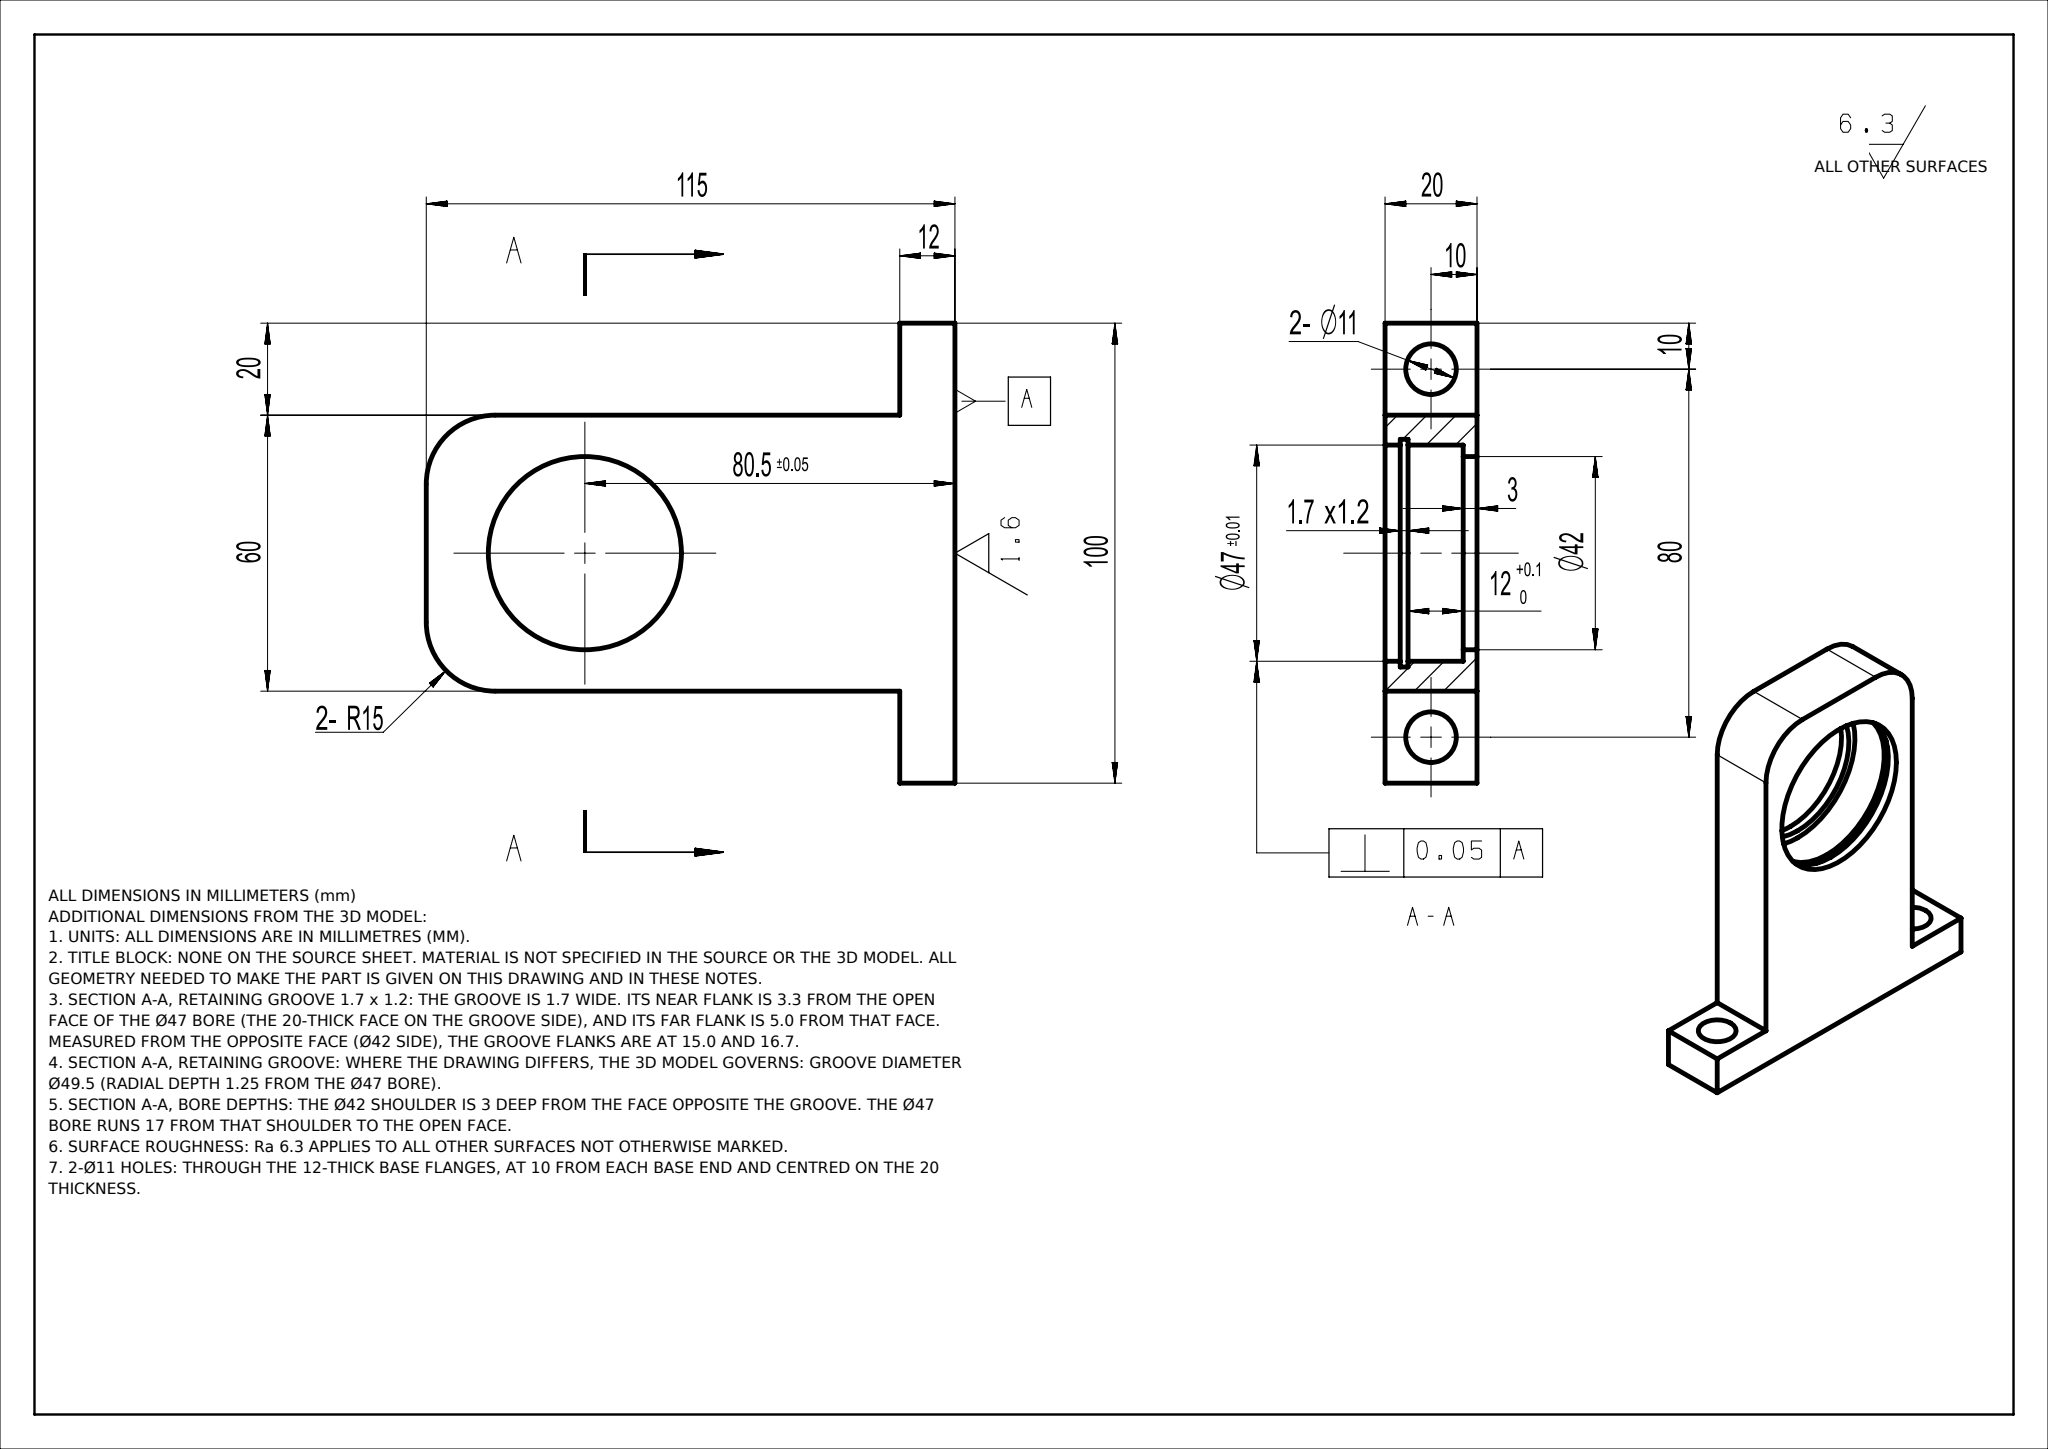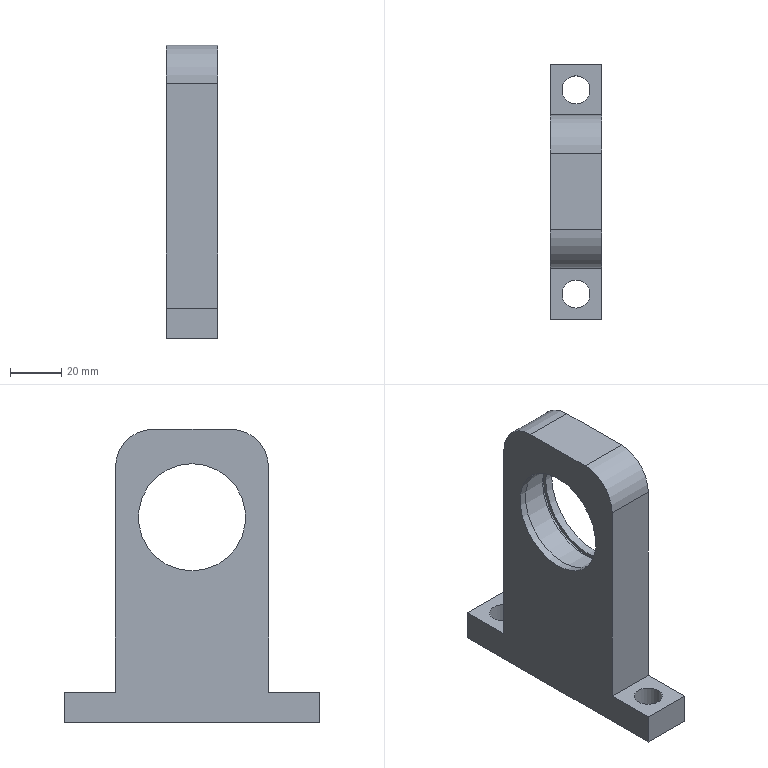Part | NX | mm | 1 solid | 21 faces | box 20 x 100 x 115 mm | volume 109415 mm3 | plane 13 | cylinder 8 | commonest cylinder face diameters 47 x2 11 x2 30 x2 42 x1 49.5 x1
STEP:
#1=CARTESIAN_POINT('',(0.,0.,0.));
#2=DIRECTION('',(0.,0.,1.));
#3=DIRECTION('',(1.,0.,0.));
#4=AXIS2_PLACEMENT_3D('',#1,#2,#3);
#5=(LENGTH_UNIT()NAMED_UNIT(*)SI_UNIT(.MILLI.,.METRE.));
#6=UNCERTAINTY_MEASURE_WITH_UNIT(LENGTH_MEASURE(0.00002),#5,'','');
#7=(NAMED_UNIT(*)PLANE_ANGLE_UNIT()SI_UNIT($,.RADIAN.));
#8=PLANE_ANGLE_MEASURE_WITH_UNIT(PLANE_ANGLE_MEASURE(0.01745),#7);
#9=DIMENSIONAL_EXPONENTS(0.,0.,0.,0.,0.,0.,0.);
#10=(CONVERSION_BASED_UNIT('',#8)NAMED_UNIT(#9)PLANE_ANGLE_UNIT());
#11=(NAMED_UNIT(*)SI_UNIT($,.STERADIAN.)SOLID_ANGLE_UNIT());
#12=(GEOMETRIC_REPRESENTATION_CONTEXT(3)GLOBAL_UNCERTAINTY_ASSIGNED_CONTEXT((#6))GLOBAL_UNIT_ASSIGNED_CONTEXT((#5,#10,#11))REPRESENTATION_CONTEXT('',''));
#13=SHAPE_REPRESENTATION('',(#4),#12);
#14=CARTESIAN_POINT('',(3.,50.,57.));
#15=VERTEX_POINT('',#14);
#16=CARTESIAN_POINT('',(3.,50.,80.5));
#17=DIRECTION('',(1.,0.,0.));
#18=DIRECTION('',(0.,0.,-1.));
#19=AXIS2_PLACEMENT_3D('',#16,#17,#18);
#20=CIRCLE('',#19,23.5);
#21=EDGE_CURVE('',#15,#15,#20,.T.);
#22=ORIENTED_EDGE('',*,*,#21,.F.);
#23=EDGE_LOOP('',(#22));
#24=FACE_BOUND('',#23,.T.);
#25=CARTESIAN_POINT('',(15.,50.,57.));
#26=VERTEX_POINT('',#25);
#27=CARTESIAN_POINT('',(15.,50.,80.5));
#28=DIRECTION('',(1.,0.,0.));
#29=DIRECTION('',(0.,0.,-1.));
#30=AXIS2_PLACEMENT_3D('',#27,#28,#29);
#31=CIRCLE('',#30,23.5);
#32=EDGE_CURVE('',#26,#26,#31,.T.);
#33=ORIENTED_EDGE('',*,*,#32,.T.);
#34=EDGE_LOOP('',(#33));
#35=FACE_BOUND('',#34,.T.);
#36=CARTESIAN_POINT('',(20.,50.,80.5));
#37=DIRECTION('',(-1.,0.,0.));
#38=DIRECTION('',(0.,0.,1.));
#39=AXIS2_PLACEMENT_3D('',#36,#37,#38);
#40=CYLINDRICAL_SURFACE('',#39,23.5);
#41=ADVANCED_FACE('',(#24,#35),#40,.F.);
#42=CARTESIAN_POINT('',(0.,-0.,0.));
#43=VERTEX_POINT('',#42);
#44=CARTESIAN_POINT('',(0.,100.,0.));
#45=VERTEX_POINT('',#44);
#46=CARTESIAN_POINT('',(0.,0.,0.));
#47=DIRECTION('',(0.,1.,0.));
#48=VECTOR('',#47,1.);
#49=LINE('',#46,#48);
#50=EDGE_CURVE('',#43,#45,#49,.T.);
#51=ORIENTED_EDGE('',*,*,#50,.T.);
#52=CARTESIAN_POINT('',(20.,100.,0.));
#53=VERTEX_POINT('',#52);
#54=CARTESIAN_POINT('',(20.,100.,0.));
#55=DIRECTION('',(-1.,0.,0.));
#56=VECTOR('',#55,1.);
#57=LINE('',#54,#56);
#58=EDGE_CURVE('',#53,#45,#57,.T.);
#59=ORIENTED_EDGE('',*,*,#58,.F.);
#60=CARTESIAN_POINT('',(20.,-0.,0.));
#61=VERTEX_POINT('',#60);
#62=CARTESIAN_POINT('',(20.,0.,0.));
#63=DIRECTION('',(0.,1.,0.));
#64=VECTOR('',#63,1.);
#65=LINE('',#62,#64);
#66=EDGE_CURVE('',#61,#53,#65,.T.);
#67=ORIENTED_EDGE('',*,*,#66,.F.);
#68=CARTESIAN_POINT('',(20.,-0.,0.));
#69=DIRECTION('',(-1.,0.,0.));
#70=VECTOR('',#69,1.);
#71=LINE('',#68,#70);
#72=EDGE_CURVE('',#61,#43,#71,.T.);
#73=ORIENTED_EDGE('',*,*,#72,.T.);
#74=EDGE_LOOP('',(#51,#59,#67,#73));
#75=FACE_BOUND('',#74,.T.);
#76=CARTESIAN_POINT('',(10.,15.5,0.));
#77=VERTEX_POINT('',#76);
#78=CARTESIAN_POINT('',(10.,10.,0.));
#79=DIRECTION('',(0.,0.,-1.));
#80=DIRECTION('',(0.,1.,0.));
#81=AXIS2_PLACEMENT_3D('',#78,#79,#80);
#82=CIRCLE('',#81,5.5);
#83=EDGE_CURVE('',#77,#77,#82,.T.);
#84=ORIENTED_EDGE('',*,*,#83,.F.);
#85=EDGE_LOOP('',(#84));
#86=FACE_BOUND('',#85,.T.);
#87=CARTESIAN_POINT('',(10.,84.5,0.));
#88=VERTEX_POINT('',#87);
#89=CARTESIAN_POINT('',(10.,90.,0.));
#90=DIRECTION('',(0.,0.,1.));
#91=DIRECTION('',(-0.,-1.,0.));
#92=AXIS2_PLACEMENT_3D('',#89,#90,#91);
#93=CIRCLE('',#92,5.5);
#94=EDGE_CURVE('',#88,#88,#93,.T.);
#95=ORIENTED_EDGE('',*,*,#94,.T.);
#96=EDGE_LOOP('',(#95));
#97=FACE_BOUND('',#96,.T.);
#98=CARTESIAN_POINT('',(20.,0.,0.));
#99=DIRECTION('',(0.,0.,1.));
#100=DIRECTION('',(1.,0.,0.));
#101=AXIS2_PLACEMENT_3D('',#98,#99,#100);
#102=PLANE('',#101);
#103=ADVANCED_FACE('',(#75,#86,#97),#102,.F.);
#104=CARTESIAN_POINT('',(0.,0.,12.));
#105=VERTEX_POINT('',#104);
#106=CARTESIAN_POINT('',(0.,0.,12.));
#107=DIRECTION('',(0.,-0.,-1.));
#108=VECTOR('',#107,1.);
#109=LINE('',#106,#108);
#110=EDGE_CURVE('',#105,#43,#109,.T.);
#111=ORIENTED_EDGE('',*,*,#110,.T.);
#112=ORIENTED_EDGE('',*,*,#72,.F.);
#113=CARTESIAN_POINT('',(20.,0.,12.));
#114=VERTEX_POINT('',#113);
#115=CARTESIAN_POINT('',(20.,0.,12.));
#116=DIRECTION('',(0.,-0.,-1.));
#117=VECTOR('',#116,1.);
#118=LINE('',#115,#117);
#119=EDGE_CURVE('',#114,#61,#118,.T.);
#120=ORIENTED_EDGE('',*,*,#119,.F.);
#121=CARTESIAN_POINT('',(20.,0.,12.));
#122=DIRECTION('',(-1.,0.,0.));
#123=VECTOR('',#122,1.);
#124=LINE('',#121,#123);
#125=EDGE_CURVE('',#114,#105,#124,.T.);
#126=ORIENTED_EDGE('',*,*,#125,.T.);
#127=EDGE_LOOP('',(#111,#112,#120,#126));
#128=FACE_OUTER_BOUND('',#127,.T.);
#129=CARTESIAN_POINT('',(20.,0.,12.));
#130=DIRECTION('',(0.,1.,-0.));
#131=DIRECTION('',(0.,0.,1.));
#132=AXIS2_PLACEMENT_3D('',#129,#130,#131);
#133=PLANE('',#132);
#134=ADVANCED_FACE('',(#128),#133,.F.);
#135=CARTESIAN_POINT('',(0.,100.,12.));
#136=VERTEX_POINT('',#135);
#137=CARTESIAN_POINT('',(0.,100.,0.));
#138=DIRECTION('',(0.,0.,1.));
#139=VECTOR('',#138,1.);
#140=LINE('',#137,#139);
#141=EDGE_CURVE('',#45,#136,#140,.T.);
#142=ORIENTED_EDGE('',*,*,#141,.T.);
#143=CARTESIAN_POINT('',(20.,100.,12.));
#144=VERTEX_POINT('',#143);
#145=CARTESIAN_POINT('',(20.,100.,12.));
#146=DIRECTION('',(-1.,0.,0.));
#147=VECTOR('',#146,1.);
#148=LINE('',#145,#147);
#149=EDGE_CURVE('',#144,#136,#148,.T.);
#150=ORIENTED_EDGE('',*,*,#149,.F.);
#151=CARTESIAN_POINT('',(20.,100.,0.));
#152=DIRECTION('',(0.,0.,1.));
#153=VECTOR('',#152,1.);
#154=LINE('',#151,#153);
#155=EDGE_CURVE('',#53,#144,#154,.T.);
#156=ORIENTED_EDGE('',*,*,#155,.F.);
#157=ORIENTED_EDGE('',*,*,#58,.T.);
#158=EDGE_LOOP('',(#142,#150,#156,#157));
#159=FACE_OUTER_BOUND('',#158,.T.);
#160=CARTESIAN_POINT('',(20.,100.,0.));
#161=DIRECTION('',(0.,-1.,0.));
#162=DIRECTION('',(0.,0.,-1.));
#163=AXIS2_PLACEMENT_3D('',#160,#161,#162);
#164=PLANE('',#163);
#165=ADVANCED_FACE('',(#159),#164,.F.);
#166=CARTESIAN_POINT('',(10.,95.5,12.));
#167=VERTEX_POINT('',#166);
#168=CARTESIAN_POINT('',(10.,90.,12.));
#169=DIRECTION('',(0.,-0.,1.));
#170=DIRECTION('',(0.,1.,0.));
#171=AXIS2_PLACEMENT_3D('',#168,#169,#170);
#172=CIRCLE('',#171,5.5);
#173=EDGE_CURVE('',#167,#167,#172,.T.);
#174=ORIENTED_EDGE('',*,*,#173,.F.);
#175=EDGE_LOOP('',(#174));
#176=FACE_BOUND('',#175,.T.);
#177=CARTESIAN_POINT('',(0.,80.,12.));
#178=VERTEX_POINT('',#177);
#179=CARTESIAN_POINT('',(0.,100.,12.));
#180=DIRECTION('',(0.,-1.,-0.));
#181=VECTOR('',#180,1.);
#182=LINE('',#179,#181);
#183=EDGE_CURVE('',#136,#178,#182,.T.);
#184=ORIENTED_EDGE('',*,*,#183,.T.);
#185=CARTESIAN_POINT('',(20.,80.,12.));
#186=VERTEX_POINT('',#185);
#187=CARTESIAN_POINT('',(20.,80.,12.));
#188=DIRECTION('',(-1.,0.,0.));
#189=VECTOR('',#188,1.);
#190=LINE('',#187,#189);
#191=EDGE_CURVE('',#186,#178,#190,.T.);
#192=ORIENTED_EDGE('',*,*,#191,.F.);
#193=CARTESIAN_POINT('',(20.,100.,12.));
#194=DIRECTION('',(0.,-1.,-0.));
#195=VECTOR('',#194,1.);
#196=LINE('',#193,#195);
#197=EDGE_CURVE('',#144,#186,#196,.T.);
#198=ORIENTED_EDGE('',*,*,#197,.F.);
#199=ORIENTED_EDGE('',*,*,#149,.T.);
#200=EDGE_LOOP('',(#184,#192,#198,#199));
#201=FACE_BOUND('',#200,.T.);
#202=CARTESIAN_POINT('',(20.,100.,12.));
#203=DIRECTION('',(0.,0.,-1.));
#204=DIRECTION('',(0.,1.,0.));
#205=AXIS2_PLACEMENT_3D('',#202,#203,#204);
#206=PLANE('',#205);
#207=ADVANCED_FACE('',(#176,#201),#206,.F.);
#208=CARTESIAN_POINT('',(0.,80.,100.));
#209=VERTEX_POINT('',#208);
#210=CARTESIAN_POINT('',(0.,80.,12.));
#211=DIRECTION('',(0.,-0.,1.));
#212=VECTOR('',#211,1.);
#213=LINE('',#210,#212);
#214=EDGE_CURVE('',#178,#209,#213,.T.);
#215=ORIENTED_EDGE('',*,*,#214,.T.);
#216=CARTESIAN_POINT('',(20.,80.,100.));
#217=VERTEX_POINT('',#216);
#218=CARTESIAN_POINT('',(20.,80.,100.));
#219=DIRECTION('',(1.,0.,0.));
#220=VECTOR('',#219,1.);
#221=LINE('',#218,#220);
#222=EDGE_CURVE('',#209,#217,#221,.T.);
#223=ORIENTED_EDGE('',*,*,#222,.T.);
#224=CARTESIAN_POINT('',(20.,80.,12.));
#225=DIRECTION('',(0.,-0.,1.));
#226=VECTOR('',#225,1.);
#227=LINE('',#224,#226);
#228=EDGE_CURVE('',#186,#217,#227,.T.);
#229=ORIENTED_EDGE('',*,*,#228,.F.);
#230=ORIENTED_EDGE('',*,*,#191,.T.);
#231=EDGE_LOOP('',(#215,#223,#229,#230));
#232=FACE_OUTER_BOUND('',#231,.T.);
#233=CARTESIAN_POINT('',(20.,80.,12.));
#234=DIRECTION('',(0.,-1.,-0.));
#235=DIRECTION('',(0.,0.,-1.));
#236=AXIS2_PLACEMENT_3D('',#233,#234,#235);
#237=PLANE('',#236);
#238=ADVANCED_FACE('',(#232),#237,.F.);
#239=CARTESIAN_POINT('',(20.,65.,115.));
#240=VERTEX_POINT('',#239);
#241=CARTESIAN_POINT('',(20.,35.,115.));
#242=VERTEX_POINT('',#241);
#243=CARTESIAN_POINT('',(20.,80.,115.));
#244=DIRECTION('',(0.,-1.,-0.));
#245=VECTOR('',#244,1.);
#246=LINE('',#243,#245);
#247=EDGE_CURVE('',#240,#242,#246,.T.);
#248=ORIENTED_EDGE('',*,*,#247,.F.);
#249=CARTESIAN_POINT('',(0.,65.,115.));
#250=VERTEX_POINT('',#249);
#251=CARTESIAN_POINT('',(20.,65.,115.));
#252=DIRECTION('',(-1.,0.,0.));
#253=VECTOR('',#252,1.);
#254=LINE('',#251,#253);
#255=EDGE_CURVE('',#240,#250,#254,.T.);
#256=ORIENTED_EDGE('',*,*,#255,.T.);
#257=CARTESIAN_POINT('',(0.,35.,115.));
#258=VERTEX_POINT('',#257);
#259=CARTESIAN_POINT('',(0.,80.,115.));
#260=DIRECTION('',(0.,-1.,-0.));
#261=VECTOR('',#260,1.);
#262=LINE('',#259,#261);
#263=EDGE_CURVE('',#250,#258,#262,.T.);
#264=ORIENTED_EDGE('',*,*,#263,.T.);
#265=CARTESIAN_POINT('',(20.,35.,115.));
#266=DIRECTION('',(1.,0.,0.));
#267=VECTOR('',#266,1.);
#268=LINE('',#265,#267);
#269=EDGE_CURVE('',#258,#242,#268,.T.);
#270=ORIENTED_EDGE('',*,*,#269,.T.);
#271=EDGE_LOOP('',(#248,#256,#264,#270));
#272=FACE_OUTER_BOUND('',#271,.T.);
#273=CARTESIAN_POINT('',(20.,80.,115.));
#274=DIRECTION('',(0.,0.,-1.));
#275=DIRECTION('',(0.,1.,0.));
#276=AXIS2_PLACEMENT_3D('',#273,#274,#275);
#277=PLANE('',#276);
#278=ADVANCED_FACE('',(#272),#277,.F.);
#279=CARTESIAN_POINT('',(20.,20.,100.));
#280=VERTEX_POINT('',#279);
#281=CARTESIAN_POINT('',(20.,20.,12.));
#282=VERTEX_POINT('',#281);
#283=CARTESIAN_POINT('',(20.,20.,115.));
#284=DIRECTION('',(0.,0.,-1.));
#285=VECTOR('',#284,1.);
#286=LINE('',#283,#285);
#287=EDGE_CURVE('',#280,#282,#286,.T.);
#288=ORIENTED_EDGE('',*,*,#287,.F.);
#289=CARTESIAN_POINT('',(0.,20.,100.));
#290=VERTEX_POINT('',#289);
#291=CARTESIAN_POINT('',(20.,20.,100.));
#292=DIRECTION('',(-1.,0.,0.));
#293=VECTOR('',#292,1.);
#294=LINE('',#291,#293);
#295=EDGE_CURVE('',#280,#290,#294,.T.);
#296=ORIENTED_EDGE('',*,*,#295,.T.);
#297=CARTESIAN_POINT('',(0.,20.,12.));
#298=VERTEX_POINT('',#297);
#299=CARTESIAN_POINT('',(0.,20.,115.));
#300=DIRECTION('',(0.,0.,-1.));
#301=VECTOR('',#300,1.);
#302=LINE('',#299,#301);
#303=EDGE_CURVE('',#290,#298,#302,.T.);
#304=ORIENTED_EDGE('',*,*,#303,.T.);
#305=CARTESIAN_POINT('',(20.,20.,12.));
#306=DIRECTION('',(-1.,0.,0.));
#307=VECTOR('',#306,1.);
#308=LINE('',#305,#307);
#309=EDGE_CURVE('',#282,#298,#308,.T.);
#310=ORIENTED_EDGE('',*,*,#309,.F.);
#311=EDGE_LOOP('',(#288,#296,#304,#310));
#312=FACE_OUTER_BOUND('',#311,.T.);
#313=CARTESIAN_POINT('',(20.,20.,115.));
#314=DIRECTION('',(0.,1.,0.));
#315=DIRECTION('',(0.,-0.,1.));
#316=AXIS2_PLACEMENT_3D('',#313,#314,#315);
#317=PLANE('',#316);
#318=ADVANCED_FACE('',(#312),#317,.F.);
#319=CARTESIAN_POINT('',(10.,15.5,12.));
#320=VERTEX_POINT('',#319);
#321=CARTESIAN_POINT('',(10.,10.,12.));
#322=DIRECTION('',(0.,0.,-1.));
#323=DIRECTION('',(0.,1.,0.));
#324=AXIS2_PLACEMENT_3D('',#321,#322,#323);
#325=CIRCLE('',#324,5.5);
#326=EDGE_CURVE('',#320,#320,#325,.T.);
#327=ORIENTED_EDGE('',*,*,#326,.T.);
#328=EDGE_LOOP('',(#327));
#329=FACE_BOUND('',#328,.T.);
#330=CARTESIAN_POINT('',(0.,20.,12.));
#331=DIRECTION('',(0.,-1.,-0.));
#332=VECTOR('',#331,1.);
#333=LINE('',#330,#332);
#334=EDGE_CURVE('',#298,#105,#333,.T.);
#335=ORIENTED_EDGE('',*,*,#334,.T.);
#336=ORIENTED_EDGE('',*,*,#125,.F.);
#337=CARTESIAN_POINT('',(20.,20.,12.));
#338=DIRECTION('',(0.,-1.,-0.));
#339=VECTOR('',#338,1.);
#340=LINE('',#337,#339);
#341=EDGE_CURVE('',#282,#114,#340,.T.);
#342=ORIENTED_EDGE('',*,*,#341,.F.);
#343=ORIENTED_EDGE('',*,*,#309,.T.);
#344=EDGE_LOOP('',(#335,#336,#342,#343));
#345=FACE_BOUND('',#344,.T.);
#346=CARTESIAN_POINT('',(20.,20.,12.));
#347=DIRECTION('',(0.,0.,-1.));
#348=DIRECTION('',(0.,1.,0.));
#349=AXIS2_PLACEMENT_3D('',#346,#347,#348);
#350=PLANE('',#349);
#351=ADVANCED_FACE('',(#329,#345),#350,.F.);
#352=CARTESIAN_POINT('',(16.7,50.,57.));
#353=VERTEX_POINT('',#352);
#354=CARTESIAN_POINT('',(16.7,50.,80.5));
#355=DIRECTION('',(1.,0.,0.));
#356=DIRECTION('',(0.,0.,-1.));
#357=AXIS2_PLACEMENT_3D('',#354,#355,#356);
#358=CIRCLE('',#357,23.5);
#359=EDGE_CURVE('',#353,#353,#358,.T.);
#360=ORIENTED_EDGE('',*,*,#359,.F.);
#361=EDGE_LOOP('',(#360));
#362=FACE_BOUND('',#361,.T.);
#363=CARTESIAN_POINT('',(20.,73.5,80.5));
#364=VERTEX_POINT('',#363);
#365=CARTESIAN_POINT('',(20.,50.,80.5));
#366=DIRECTION('',(1.,0.,0.));
#367=DIRECTION('',(0.,1.,0.));
#368=AXIS2_PLACEMENT_3D('',#365,#366,#367);
#369=CIRCLE('',#368,23.5);
#370=EDGE_CURVE('',#364,#364,#369,.T.);
#371=ORIENTED_EDGE('',*,*,#370,.T.);
#372=EDGE_LOOP('',(#371));
#373=FACE_BOUND('',#372,.T.);
#374=CARTESIAN_POINT('',(20.,50.,80.5));
#375=DIRECTION('',(-1.,0.,0.));
#376=DIRECTION('',(0.,0.,1.));
#377=AXIS2_PLACEMENT_3D('',#374,#375,#376);
#378=CYLINDRICAL_SURFACE('',#377,23.5);
#379=ADVANCED_FACE('',(#362,#373),#378,.F.);
#380=ORIENTED_EDGE('',*,*,#228,.T.);
#381=CARTESIAN_POINT('',(20.,65.,100.));
#382=DIRECTION('',(1.,0.,0.));
#383=DIRECTION('',(0.,0.,-1.));
#384=AXIS2_PLACEMENT_3D('',#381,#382,#383);
#385=CIRCLE('',#384,15.);
#386=EDGE_CURVE('',#217,#240,#385,.T.);
#387=ORIENTED_EDGE('',*,*,#386,.T.);
#388=ORIENTED_EDGE('',*,*,#247,.T.);
#389=CARTESIAN_POINT('',(20.,35.,100.));
#390=DIRECTION('',(1.,0.,0.));
#391=DIRECTION('',(0.,0.,-1.));
#392=AXIS2_PLACEMENT_3D('',#389,#390,#391);
#393=CIRCLE('',#392,15.);
#394=EDGE_CURVE('',#242,#280,#393,.T.);
#395=ORIENTED_EDGE('',*,*,#394,.T.);
#396=ORIENTED_EDGE('',*,*,#287,.T.);
#397=ORIENTED_EDGE('',*,*,#341,.T.);
#398=ORIENTED_EDGE('',*,*,#119,.T.);
#399=ORIENTED_EDGE('',*,*,#66,.T.);
#400=ORIENTED_EDGE('',*,*,#155,.T.);
#401=ORIENTED_EDGE('',*,*,#197,.T.);
#402=EDGE_LOOP('',(#380,#387,#388,#395,#396,#397,#398,#399,#400,#401));
#403=FACE_BOUND('',#402,.T.);
#404=ORIENTED_EDGE('',*,*,#370,.F.);
#405=EDGE_LOOP('',(#404));
#406=FACE_BOUND('',#405,.T.);
#407=CARTESIAN_POINT('',(20.,50.,80.5));
#408=DIRECTION('',(1.,0.,0.));
#409=DIRECTION('',(0.,0.,-1.));
#410=AXIS2_PLACEMENT_3D('',#407,#408,#409);
#411=PLANE('',#410);
#412=ADVANCED_FACE('',(#403,#406),#411,.T.);
#413=ORIENTED_EDGE('',*,*,#263,.F.);
#414=CARTESIAN_POINT('',(0.,65.,100.));
#415=DIRECTION('',(-1.,0.,0.));
#416=DIRECTION('',(0.,0.,-1.));
#417=AXIS2_PLACEMENT_3D('',#414,#415,#416);
#418=CIRCLE('',#417,15.);
#419=EDGE_CURVE('',#250,#209,#418,.T.);
#420=ORIENTED_EDGE('',*,*,#419,.T.);
#421=ORIENTED_EDGE('',*,*,#214,.F.);
#422=ORIENTED_EDGE('',*,*,#183,.F.);
#423=ORIENTED_EDGE('',*,*,#141,.F.);
#424=ORIENTED_EDGE('',*,*,#50,.F.);
#425=ORIENTED_EDGE('',*,*,#110,.F.);
#426=ORIENTED_EDGE('',*,*,#334,.F.);
#427=ORIENTED_EDGE('',*,*,#303,.F.);
#428=CARTESIAN_POINT('',(0.,35.,100.));
#429=DIRECTION('',(-1.,0.,0.));
#430=DIRECTION('',(0.,0.,-1.));
#431=AXIS2_PLACEMENT_3D('',#428,#429,#430);
#432=CIRCLE('',#431,15.);
#433=EDGE_CURVE('',#290,#258,#432,.T.);
#434=ORIENTED_EDGE('',*,*,#433,.T.);
#435=EDGE_LOOP('',(#413,#420,#421,#422,#423,#424,#425,#426,#427,#434));
#436=FACE_BOUND('',#435,.T.);
#437=CARTESIAN_POINT('',(0.,50.,59.5));
#438=VERTEX_POINT('',#437);
#439=CARTESIAN_POINT('',(0.,50.,80.5));
#440=DIRECTION('',(-1.,0.,0.));
#441=DIRECTION('',(0.,0.,-1.));
#442=AXIS2_PLACEMENT_3D('',#439,#440,#441);
#443=CIRCLE('',#442,21.);
#444=EDGE_CURVE('',#438,#438,#443,.T.);
#445=ORIENTED_EDGE('',*,*,#444,.F.);
#446=EDGE_LOOP('',(#445));
#447=FACE_BOUND('',#446,.T.);
#448=CARTESIAN_POINT('',(0.,50.,80.5));
#449=DIRECTION('',(1.,0.,0.));
#450=DIRECTION('',(0.,0.,-1.));
#451=AXIS2_PLACEMENT_3D('',#448,#449,#450);
#452=PLANE('',#451);
#453=ADVANCED_FACE('',(#436,#447),#452,.F.);
#454=ORIENTED_EDGE('',*,*,#83,.T.);
#455=EDGE_LOOP('',(#454));
#456=FACE_BOUND('',#455,.T.);
#457=ORIENTED_EDGE('',*,*,#326,.F.);
#458=EDGE_LOOP('',(#457));
#459=FACE_BOUND('',#458,.T.);
#460=CARTESIAN_POINT('',(10.,10.,20.));
#461=DIRECTION('',(0.,0.,-1.));
#462=DIRECTION('',(-1.,0.,0.));
#463=AXIS2_PLACEMENT_3D('',#460,#461,#462);
#464=CYLINDRICAL_SURFACE('',#463,5.5);
#465=ADVANCED_FACE('',(#456,#459),#464,.F.);
#466=ORIENTED_EDGE('',*,*,#94,.F.);
#467=EDGE_LOOP('',(#466));
#468=FACE_BOUND('',#467,.T.);
#469=ORIENTED_EDGE('',*,*,#173,.T.);
#470=EDGE_LOOP('',(#469));
#471=FACE_BOUND('',#470,.T.);
#472=CARTESIAN_POINT('',(10.,90.,20.));
#473=DIRECTION('',(0.,0.,-1.));
#474=DIRECTION('',(-1.,0.,0.));
#475=AXIS2_PLACEMENT_3D('',#472,#473,#474);
#476=CYLINDRICAL_SURFACE('',#475,5.5);
#477=ADVANCED_FACE('',(#468,#471),#476,.F.);
#478=ORIENTED_EDGE('',*,*,#386,.F.);
#479=ORIENTED_EDGE('',*,*,#222,.F.);
#480=ORIENTED_EDGE('',*,*,#419,.F.);
#481=ORIENTED_EDGE('',*,*,#255,.F.);
#482=EDGE_LOOP('',(#478,#479,#480,#481));
#483=FACE_OUTER_BOUND('',#482,.T.);
#484=CARTESIAN_POINT('',(20.,65.,100.));
#485=DIRECTION('',(-1.,0.,0.));
#486=DIRECTION('',(0.,0.,1.));
#487=AXIS2_PLACEMENT_3D('',#484,#485,#486);
#488=CYLINDRICAL_SURFACE('',#487,15.);
#489=ADVANCED_FACE('',(#483),#488,.T.);
#490=ORIENTED_EDGE('',*,*,#394,.F.);
#491=ORIENTED_EDGE('',*,*,#269,.F.);
#492=ORIENTED_EDGE('',*,*,#433,.F.);
#493=ORIENTED_EDGE('',*,*,#295,.F.);
#494=EDGE_LOOP('',(#490,#491,#492,#493));
#495=FACE_OUTER_BOUND('',#494,.T.);
#496=CARTESIAN_POINT('',(20.,35.,100.));
#497=DIRECTION('',(-1.,0.,0.));
#498=DIRECTION('',(0.,0.,1.));
#499=AXIS2_PLACEMENT_3D('',#496,#497,#498);
#500=CYLINDRICAL_SURFACE('',#499,15.);
#501=ADVANCED_FACE('',(#495),#500,.T.);
#502=CARTESIAN_POINT('',(3.,50.,59.5));
#503=VERTEX_POINT('',#502);
#504=CARTESIAN_POINT('',(3.,50.,80.5));
#505=DIRECTION('',(-1.,0.,0.));
#506=DIRECTION('',(0.,0.,-1.));
#507=AXIS2_PLACEMENT_3D('',#504,#505,#506);
#508=CIRCLE('',#507,21.);
#509=EDGE_CURVE('',#503,#503,#508,.T.);
#510=ORIENTED_EDGE('',*,*,#509,.T.);
#511=EDGE_LOOP('',(#510));
#512=FACE_BOUND('',#511,.T.);
#513=ORIENTED_EDGE('',*,*,#21,.T.);
#514=EDGE_LOOP('',(#513));
#515=FACE_BOUND('',#514,.T.);
#516=CARTESIAN_POINT('',(3.,50.,80.5));
#517=DIRECTION('',(1.,0.,0.));
#518=DIRECTION('',(0.,0.,-1.));
#519=AXIS2_PLACEMENT_3D('',#516,#517,#518);
#520=PLANE('',#519);
#521=ADVANCED_FACE('',(#512,#515),#520,.T.);
#522=ORIENTED_EDGE('',*,*,#444,.T.);
#523=EDGE_LOOP('',(#522));
#524=FACE_BOUND('',#523,.T.);
#525=ORIENTED_EDGE('',*,*,#509,.F.);
#526=EDGE_LOOP('',(#525));
#527=FACE_BOUND('',#526,.T.);
#528=CARTESIAN_POINT('',(0.,50.,80.5));
#529=DIRECTION('',(1.,0.,0.));
#530=DIRECTION('',(0.,0.,-1.));
#531=AXIS2_PLACEMENT_3D('',#528,#529,#530);
#532=CYLINDRICAL_SURFACE('',#531,21.);
#533=ADVANCED_FACE('',(#524,#527),#532,.F.);
#534=CARTESIAN_POINT('',(16.7,50.,55.75));
#535=VERTEX_POINT('',#534);
#536=CARTESIAN_POINT('',(16.7,50.,80.5));
#537=DIRECTION('',(-1.,0.,0.));
#538=DIRECTION('',(0.,0.,-1.));
#539=AXIS2_PLACEMENT_3D('',#536,#537,#538);
#540=CIRCLE('',#539,24.75);
#541=EDGE_CURVE('',#535,#535,#540,.T.);
#542=ORIENTED_EDGE('',*,*,#541,.F.);
#543=EDGE_LOOP('',(#542));
#544=FACE_BOUND('',#543,.T.);
#545=CARTESIAN_POINT('',(15.,50.,55.75));
#546=VERTEX_POINT('',#545);
#547=CARTESIAN_POINT('',(15.,50.,80.5));
#548=DIRECTION('',(-1.,0.,0.));
#549=DIRECTION('',(0.,0.,-1.));
#550=AXIS2_PLACEMENT_3D('',#547,#548,#549);
#551=CIRCLE('',#550,24.75);
#552=EDGE_CURVE('',#546,#546,#551,.T.);
#553=ORIENTED_EDGE('',*,*,#552,.T.);
#554=EDGE_LOOP('',(#553));
#555=FACE_BOUND('',#554,.T.);
#556=CARTESIAN_POINT('',(15.85,50.,80.5));
#557=DIRECTION('',(1.,0.,0.));
#558=DIRECTION('',(0.,0.,-1.));
#559=AXIS2_PLACEMENT_3D('',#556,#557,#558);
#560=CYLINDRICAL_SURFACE('',#559,24.75);
#561=ADVANCED_FACE('',(#544,#555),#560,.F.);
#562=ORIENTED_EDGE('',*,*,#32,.F.);
#563=EDGE_LOOP('',(#562));
#564=FACE_BOUND('',#563,.T.);
#565=ORIENTED_EDGE('',*,*,#552,.F.);
#566=EDGE_LOOP('',(#565));
#567=FACE_BOUND('',#566,.T.);
#568=CARTESIAN_POINT('',(15.,50.,80.5));
#569=DIRECTION('',(1.,0.,0.));
#570=DIRECTION('',(0.,0.,-1.));
#571=AXIS2_PLACEMENT_3D('',#568,#569,#570);
#572=PLANE('',#571);
#573=ADVANCED_FACE('',(#564,#567),#572,.T.);
#574=ORIENTED_EDGE('',*,*,#359,.T.);
#575=EDGE_LOOP('',(#574));
#576=FACE_BOUND('',#575,.T.);
#577=ORIENTED_EDGE('',*,*,#541,.T.);
#578=EDGE_LOOP('',(#577));
#579=FACE_BOUND('',#578,.T.);
#580=CARTESIAN_POINT('',(16.7,50.,80.5));
#581=DIRECTION('',(1.,0.,0.));
#582=DIRECTION('',(0.,0.,-1.));
#583=AXIS2_PLACEMENT_3D('',#580,#581,#582);
#584=PLANE('',#583);
#585=ADVANCED_FACE('',(#576,#579),#584,.F.);
#586=CLOSED_SHELL('',(#41,#103,#134,#165,#207,#238,#278,#318,#351,#379,#412,#453,#465,#477,#489,#501,#521,#533,#561,#573,#585));
#587=MANIFOLD_SOLID_BREP('',#586);
#588=ADVANCED_BREP_SHAPE_REPRESENTATION('',(#587),#12);
#589=SHAPE_REPRESENTATION_RELATIONSHIP('','',#13,#588);
#590=PRESENTATION_LAYER_ASSIGNMENT('','',(#587));
#591=COLOUR_RGB('',0.8,0.8,0.8);
#592=FILL_AREA_STYLE_COLOUR('',#591);
#593=FILL_AREA_STYLE('',(#592));
#594=SURFACE_STYLE_FILL_AREA(#593);
#595=SURFACE_SIDE_STYLE('',(#594));
#596=SURFACE_STYLE_USAGE(.BOTH.,#595);
#597=PRESENTATION_STYLE_ASSIGNMENT((#596));
#598=STYLED_ITEM('',(#597),#587);
#599=MECHANICAL_DESIGN_GEOMETRIC_PRESENTATION_REPRESENTATION('',(#598),#12);